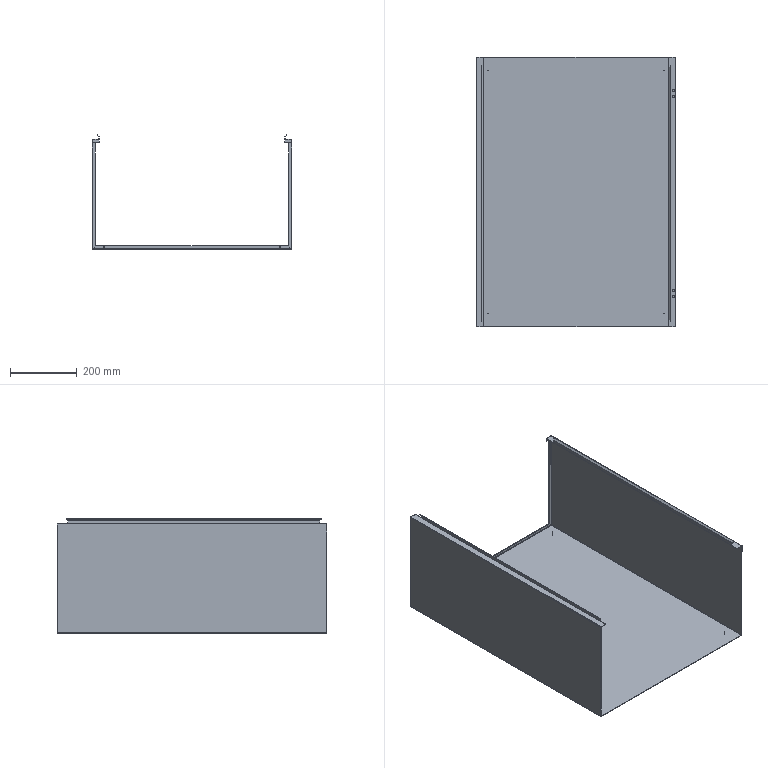Component | SolidWorks | Box-1 | 1 solid | 148 faces | volume 1625717 mm3 | plane 98 | cylinder 42 | spline 8 | commonest cylinder face diameters 3.2 x13 0.2 x13 7 x8 2 x8